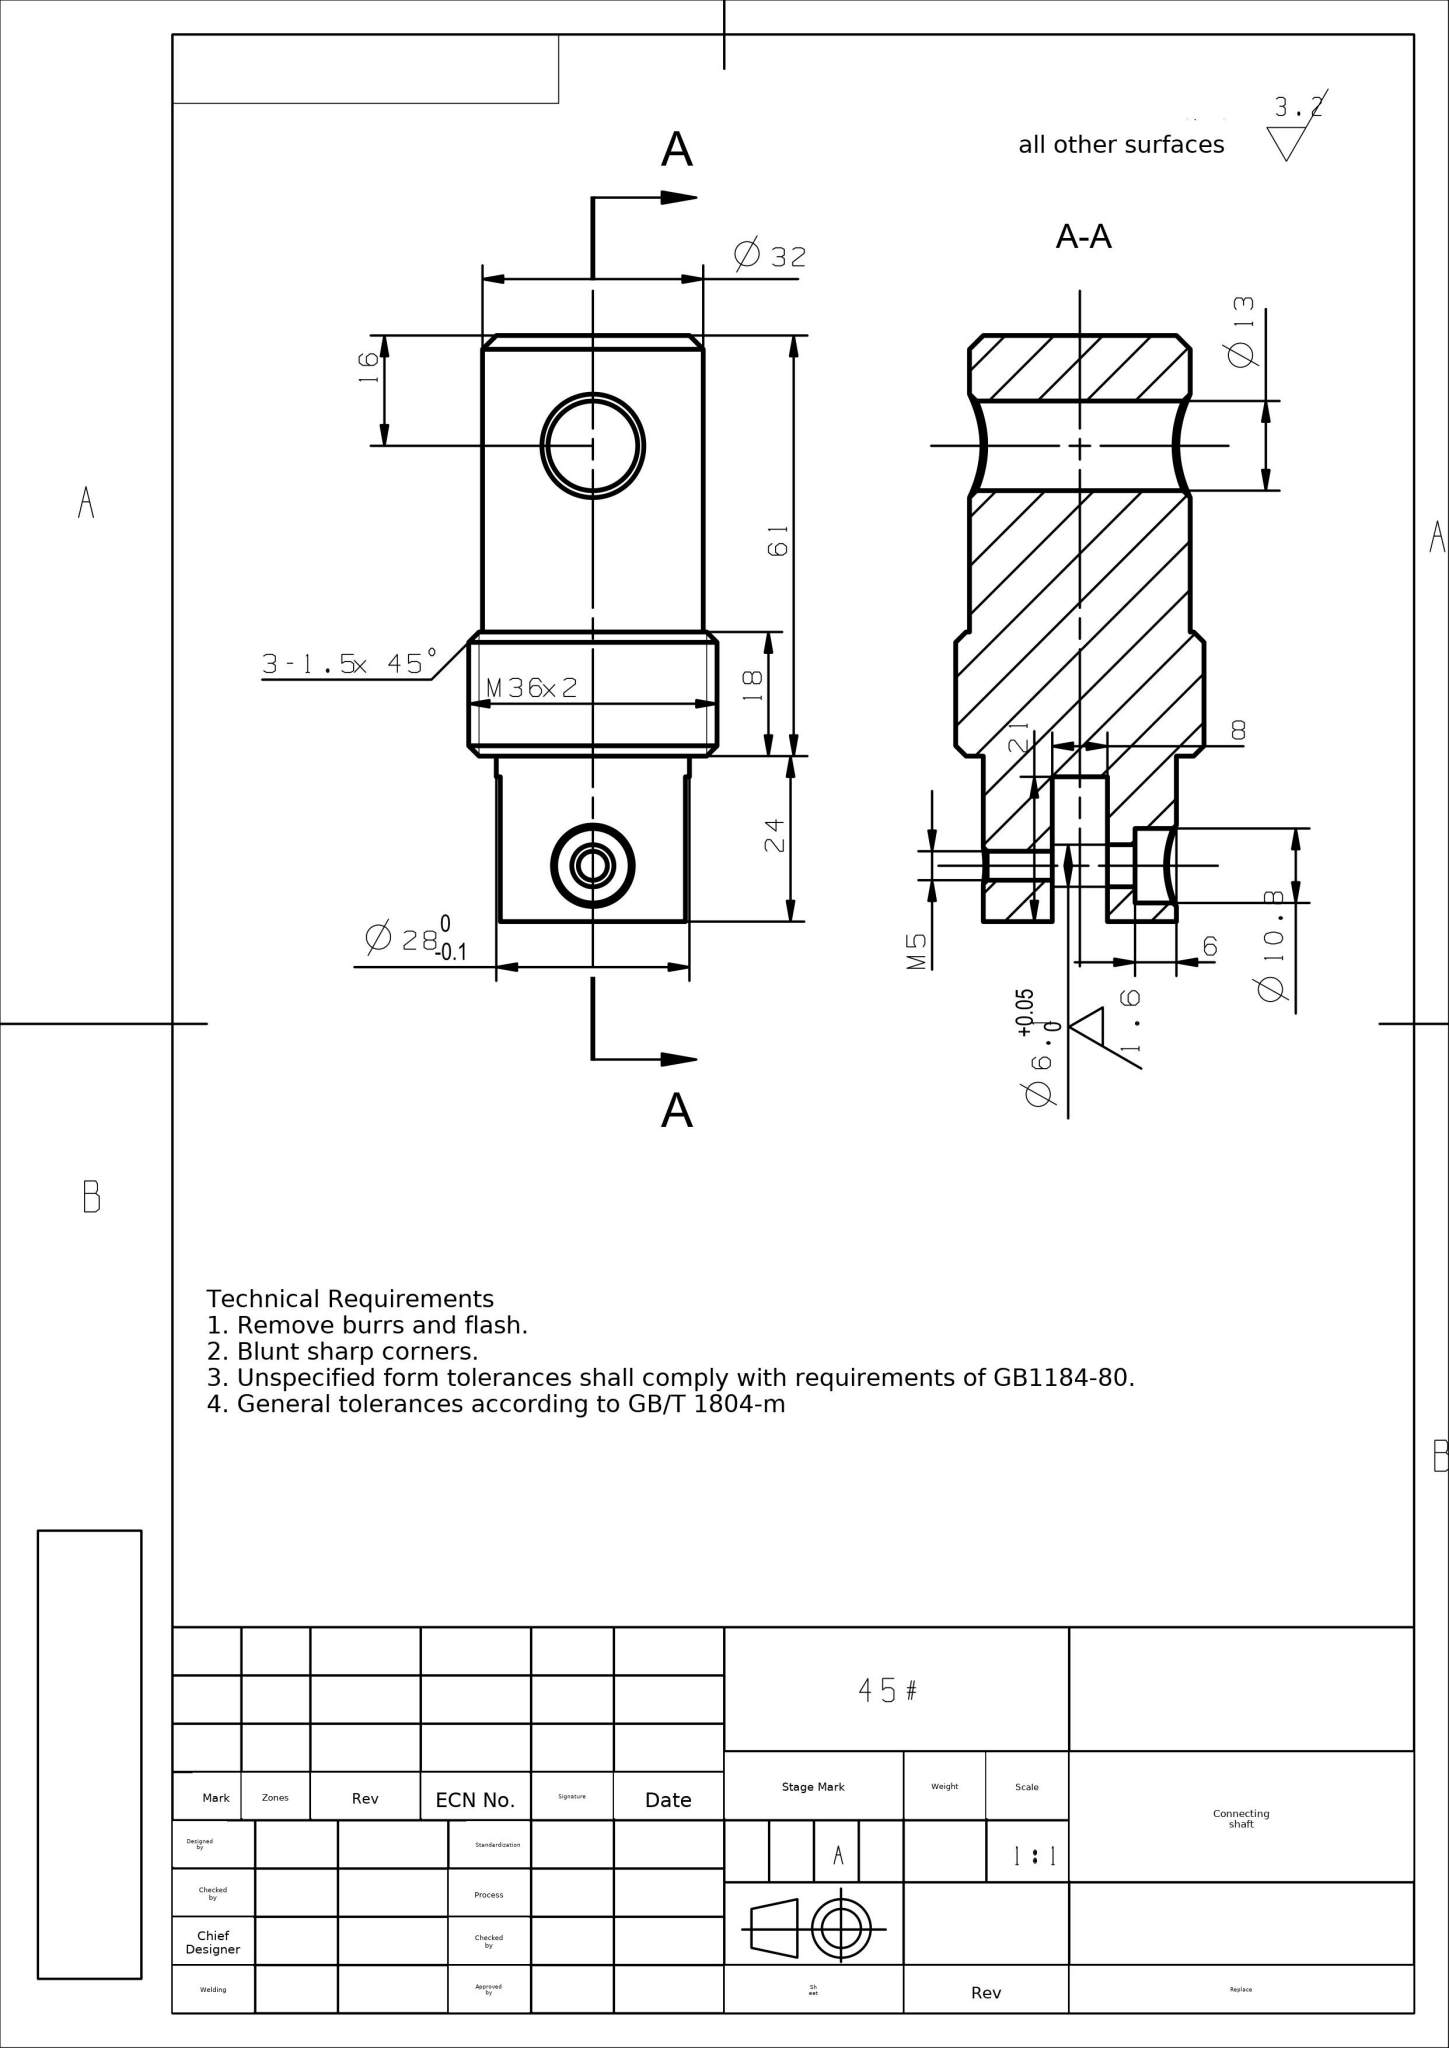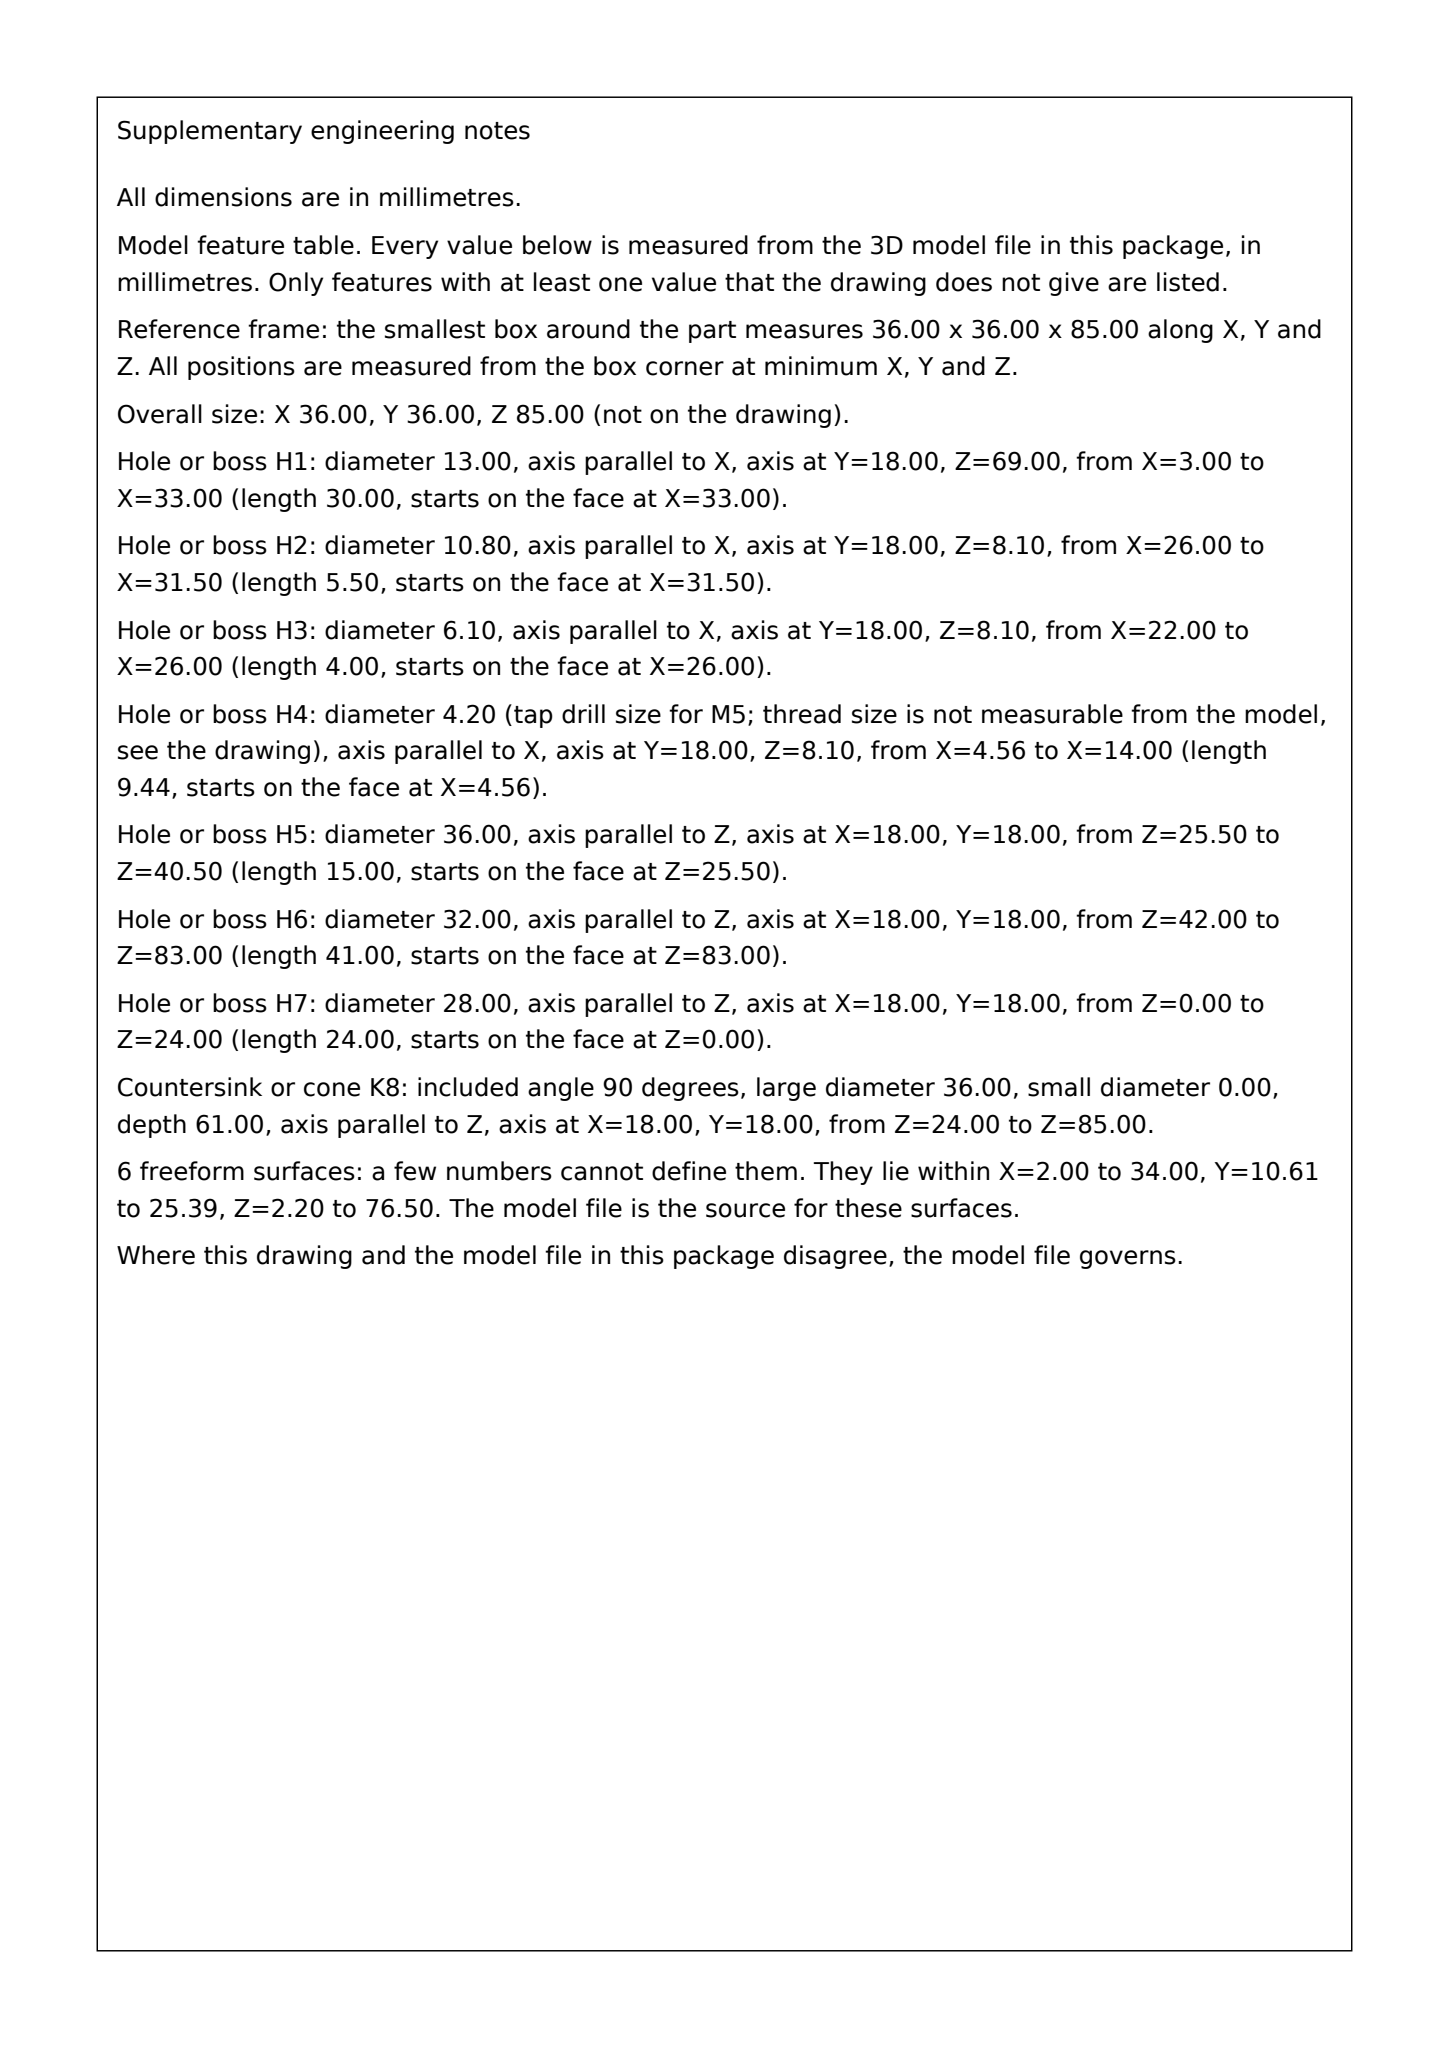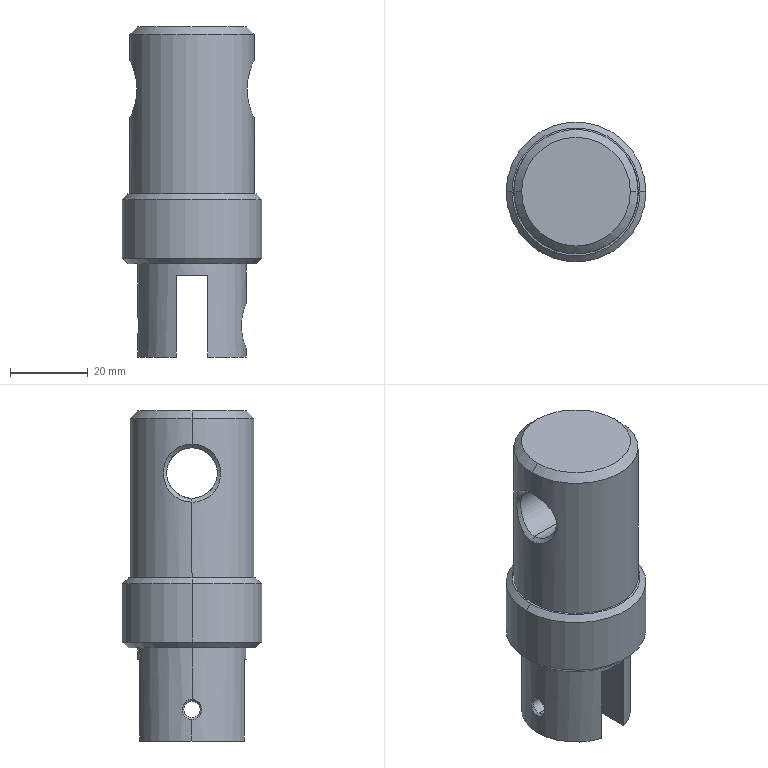Part | SolidWorks | mm | material 45# | 1 solid | 37 faces | box 36 x 36 x 85 mm | volume 57620 mm3 | cylinder 14 | plane 9 | cone 8 | spline 6 | commonest cylinder face diameters 32 x2 6.1 x2 28 x2 36 x2 4.2 x2 10.8 x2 13 x2